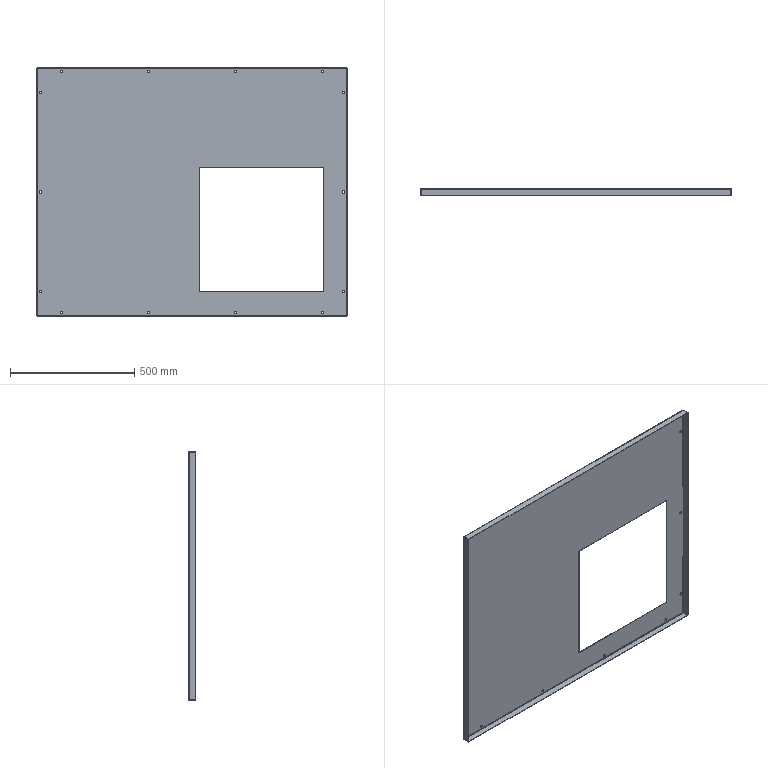Component | SolidWorks | 42TopPlateII-1 | 1 solid | 70 faces | volume 2223152 mm3 | cylinder 36 | plane 26 | spline 8 | commonest cylinder face diameters 10 x28 2 x4 6 x4